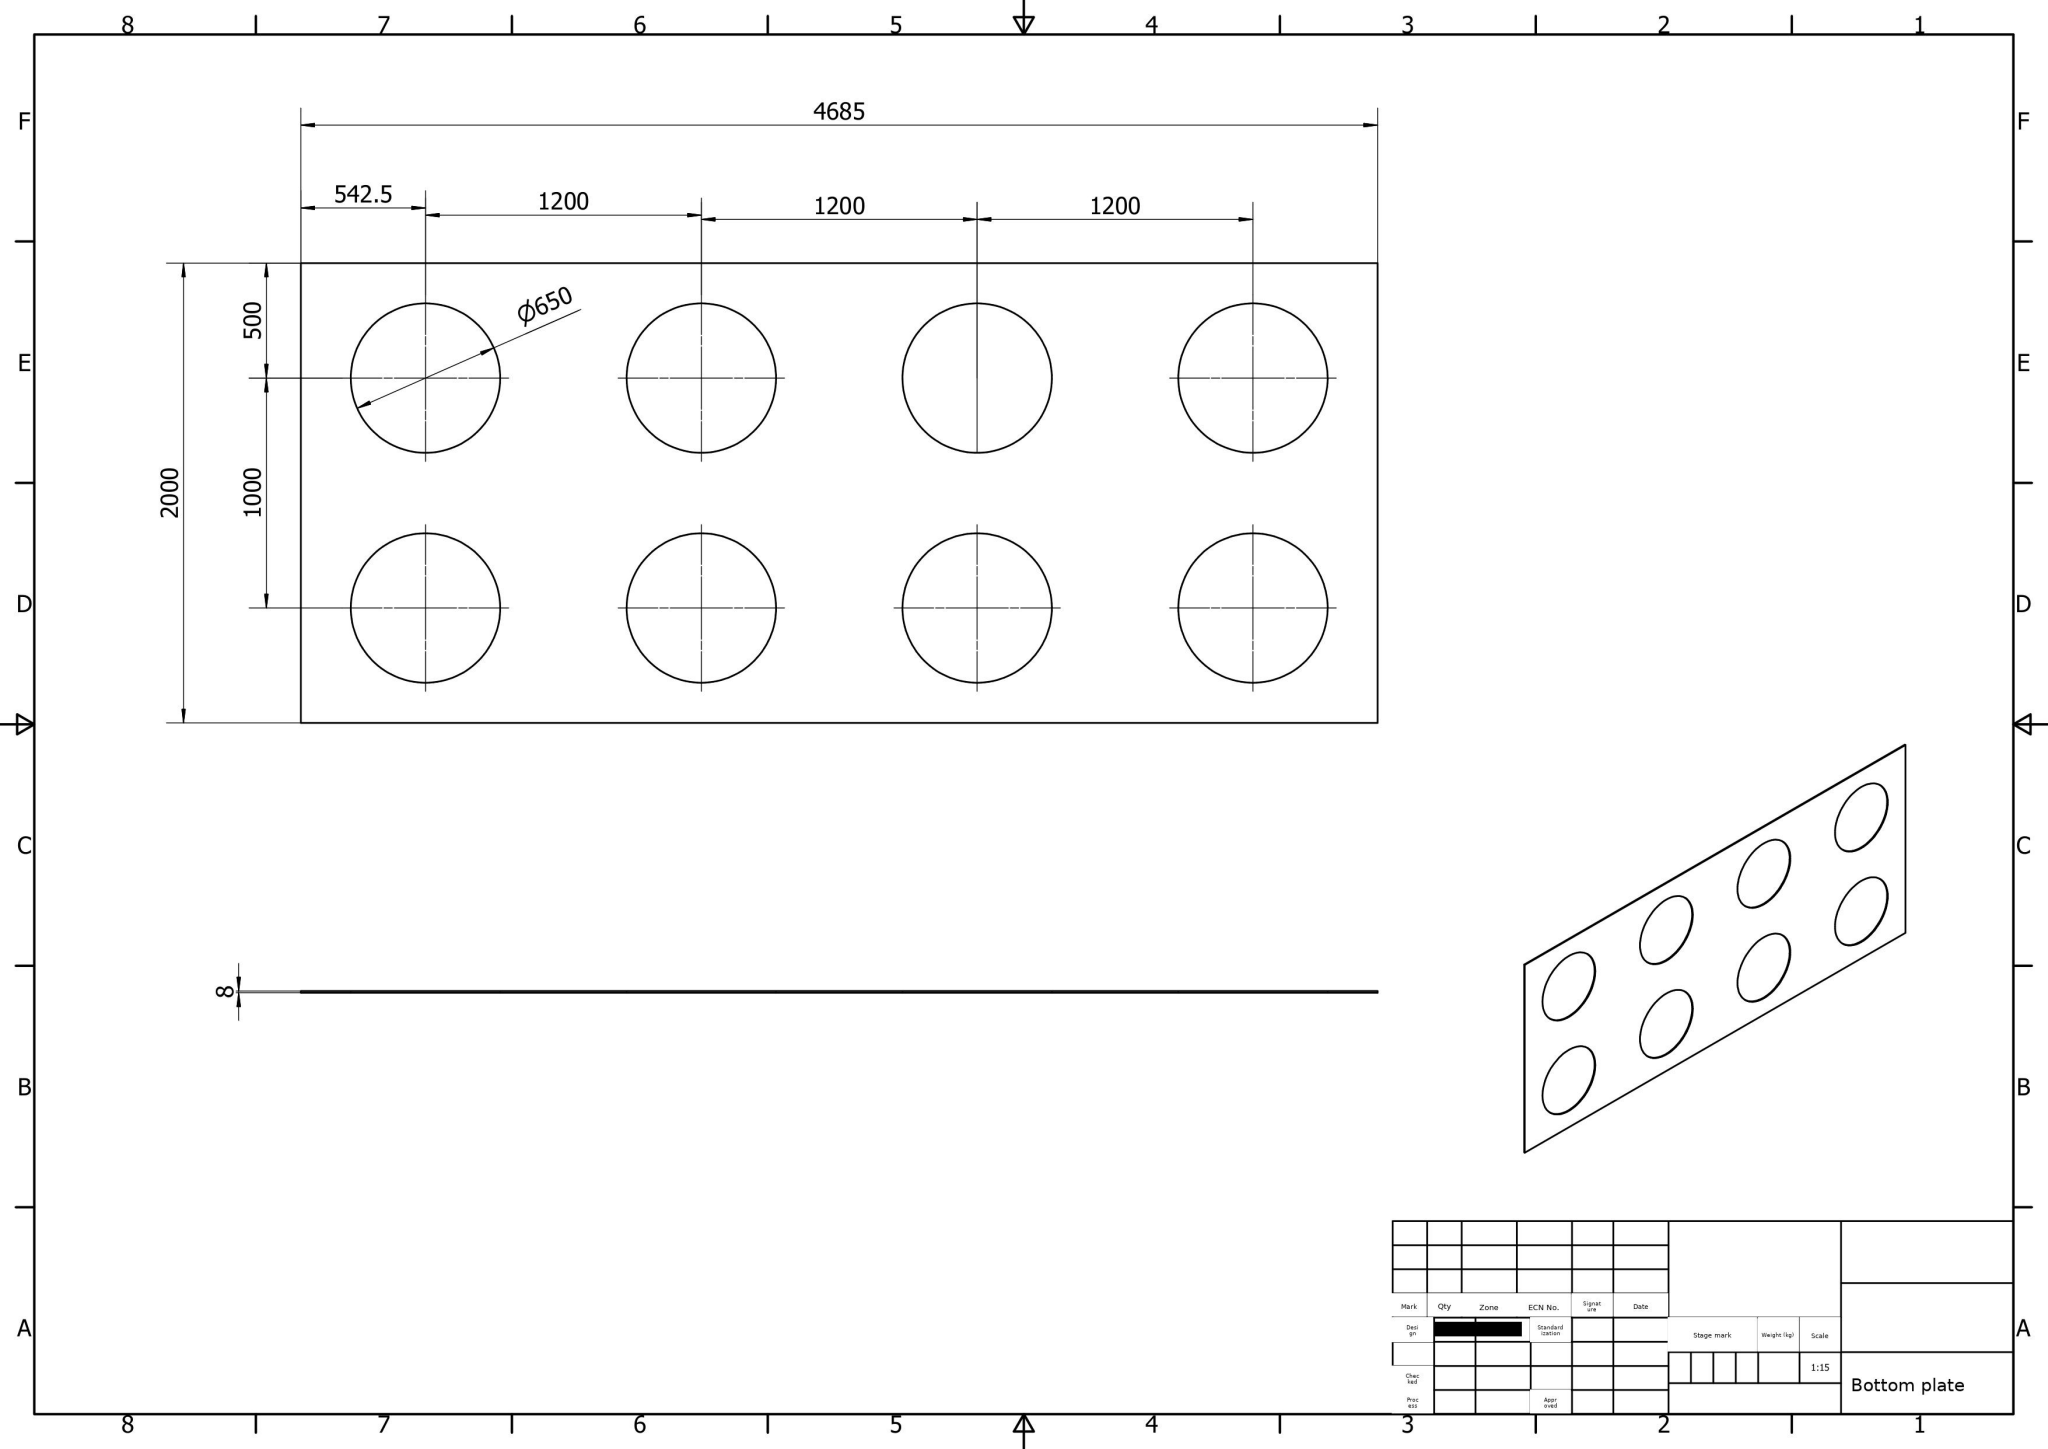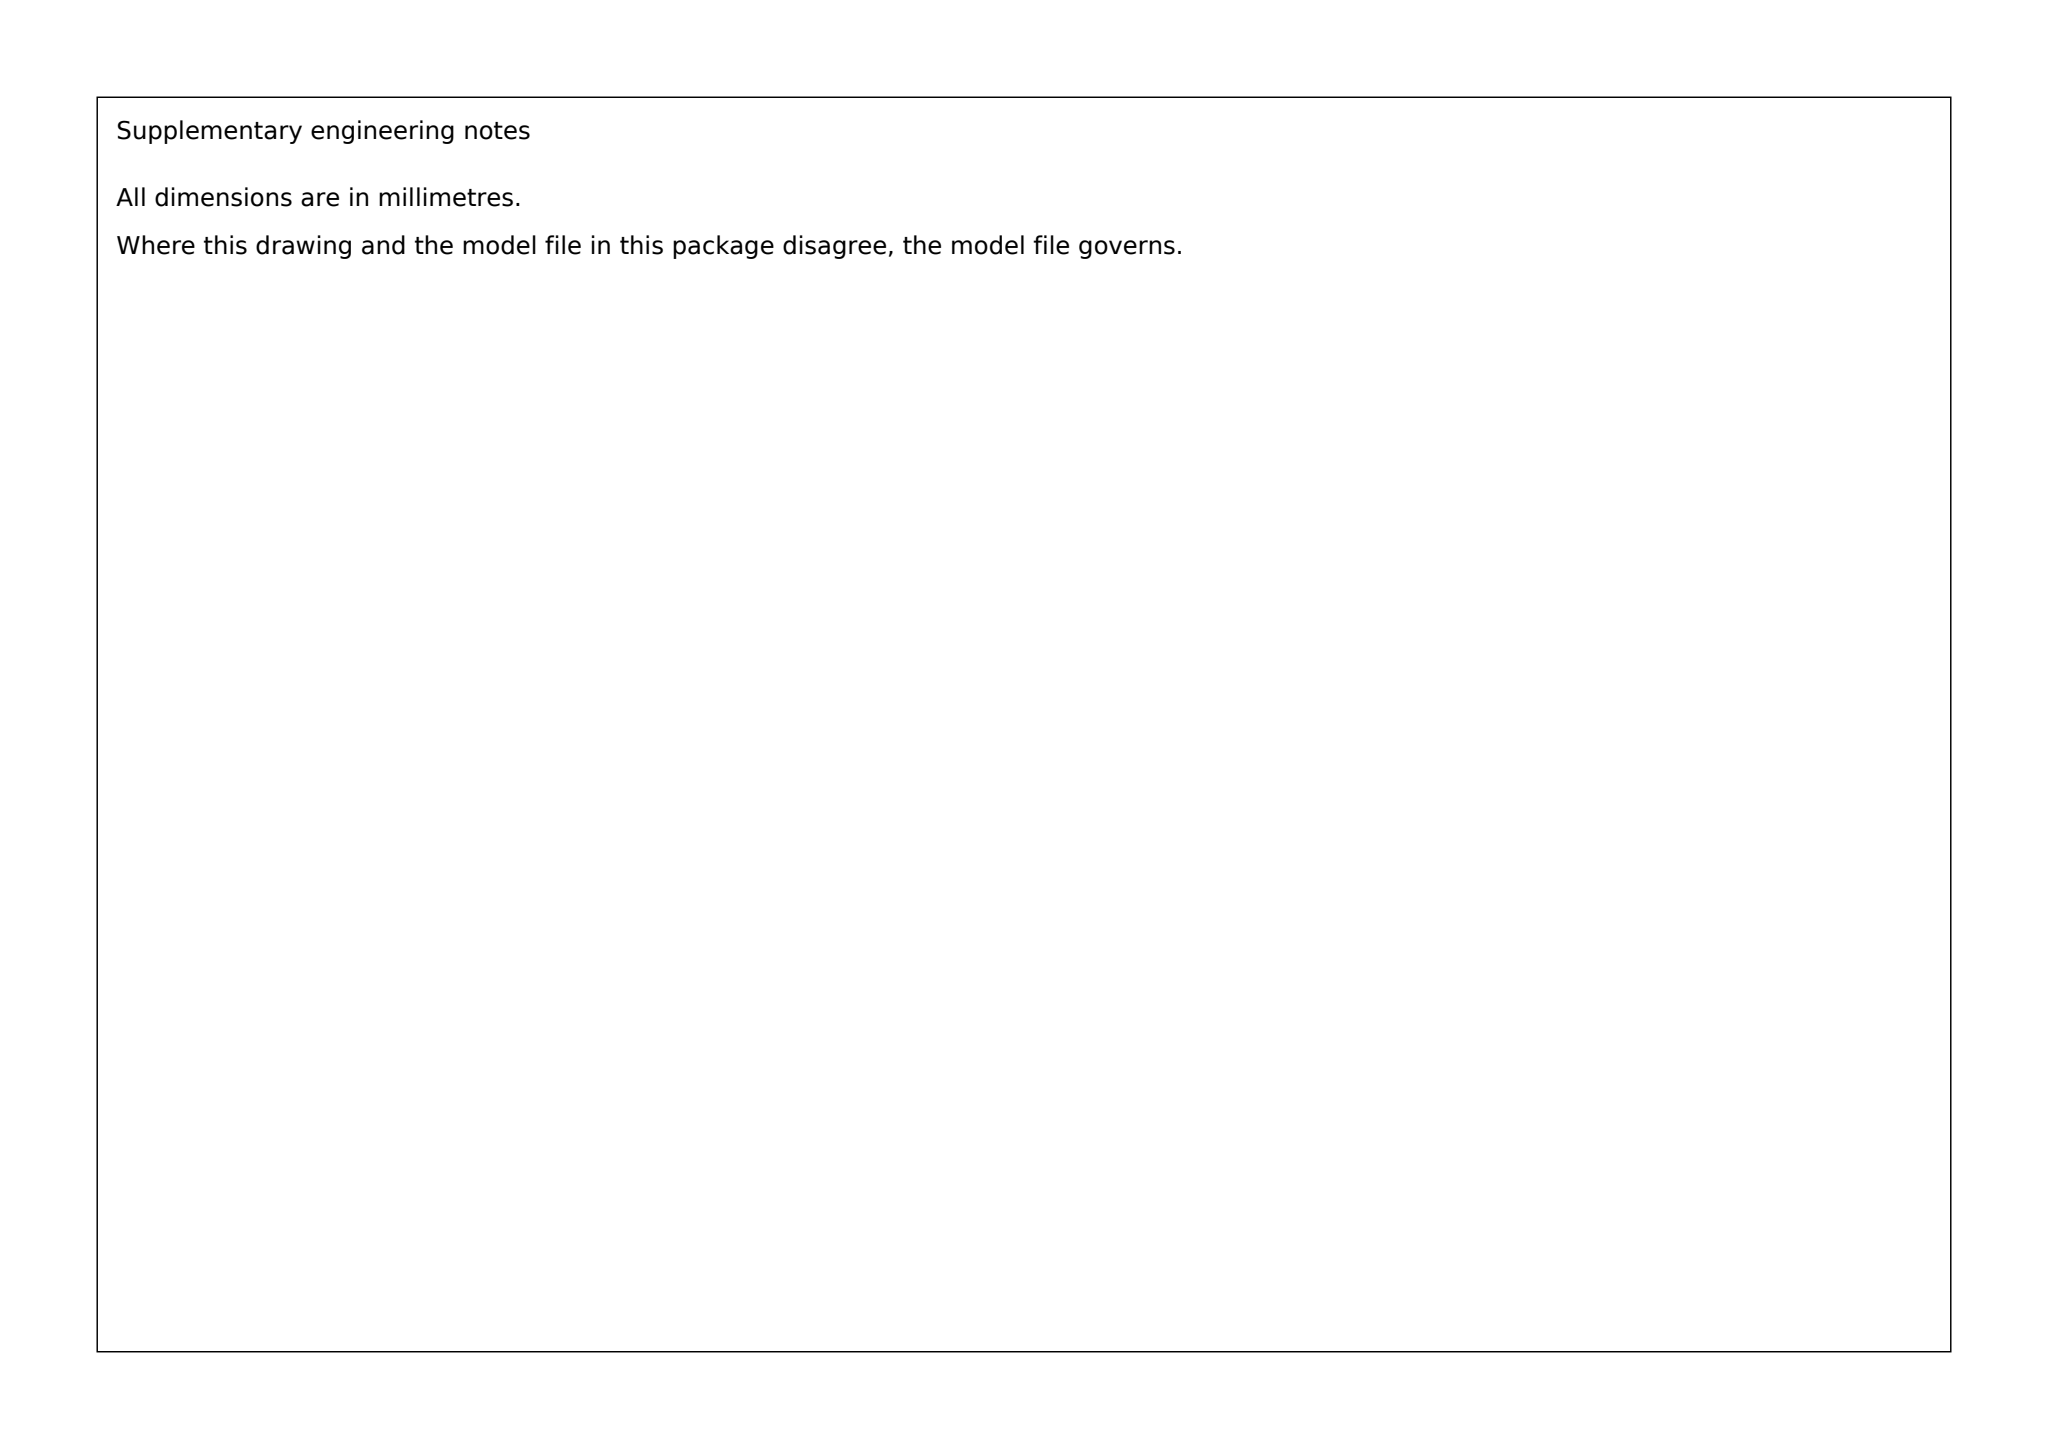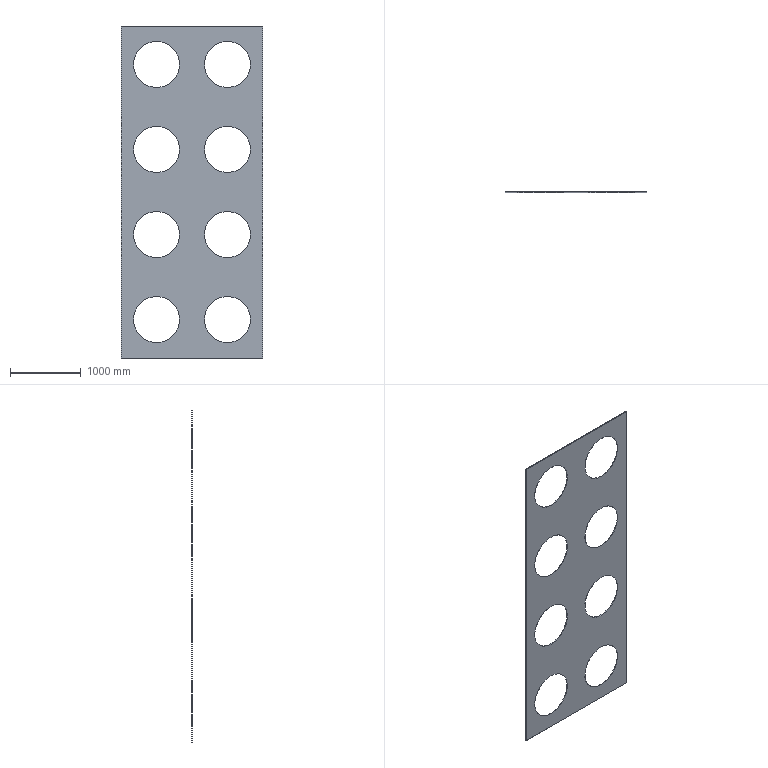Part | SolidWorks | mm | 1 solid | 22 faces | box 2000 x 8 x 4685 mm | volume 53722834 mm3 | cylinder 16 | plane 6 | commonest cylinder face diameters 650 x16
STEP:
#1=CARTESIAN_POINT('',(-500.,8.,2125.));
#2=VERTEX_POINT('',#1);
#3=CARTESIAN_POINT('',(-500.,8.,1475.));
#4=VERTEX_POINT('',#3);
#5=CARTESIAN_POINT('',(-500.,8.,1800.));
#6=DIRECTION('',(0.,-1.,0.));
#7=DIRECTION('',(0.,0.,-1.));
#8=AXIS2_PLACEMENT_3D('',#5,#6,#7);
#9=CIRCLE('',#8,325.);
#10=EDGE_CURVE('',#2,#4,#9,.T.);
#11=ORIENTED_EDGE('',*,*,#10,.F.);
#12=CARTESIAN_POINT('',(-500.,0.,2125.));
#13=VERTEX_POINT('',#12);
#14=CARTESIAN_POINT('',(-500.,8.,2125.));
#15=DIRECTION('',(0.,-1.,0.));
#16=VECTOR('',#15,1000.);
#17=LINE('',#14,#16);
#18=EDGE_CURVE('',#2,#13,#17,.T.);
#19=ORIENTED_EDGE('',*,*,#18,.T.);
#20=CARTESIAN_POINT('',(-500.,0.,1475.));
#21=VERTEX_POINT('',#20);
#22=CARTESIAN_POINT('',(-500.,0.,1800.));
#23=DIRECTION('',(0.,1.,0.));
#24=DIRECTION('',(0.,0.,-1.));
#25=AXIS2_PLACEMENT_3D('',#22,#23,#24);
#26=CIRCLE('',#25,325.);
#27=EDGE_CURVE('',#21,#13,#26,.T.);
#28=ORIENTED_EDGE('',*,*,#27,.F.);
#29=CARTESIAN_POINT('',(-500.,8.,1475.));
#30=DIRECTION('',(0.,-1.,0.));
#31=VECTOR('',#30,1000.);
#32=LINE('',#29,#31);
#33=EDGE_CURVE('',#4,#21,#32,.T.);
#34=ORIENTED_EDGE('',*,*,#33,.F.);
#35=EDGE_LOOP('',(#11,#19,#28,#34));
#36=FACE_OUTER_BOUND('',#35,.T.);
#37=CARTESIAN_POINT('',(-500.,8.,1800.));
#38=DIRECTION('',(0.,-1.,0.));
#39=DIRECTION('',(0.,0.,-1.));
#40=AXIS2_PLACEMENT_3D('',#37,#38,#39);
#41=CYLINDRICAL_SURFACE('',#40,325.);
#42=ADVANCED_FACE('',(#36),#41,.F.);
#43=CARTESIAN_POINT('',(-500.,8.,-1475.));
#44=VERTEX_POINT('',#43);
#45=CARTESIAN_POINT('',(-500.,8.,-2125.));
#46=VERTEX_POINT('',#45);
#47=CARTESIAN_POINT('',(-500.,8.,-1800.));
#48=DIRECTION('',(0.,-1.,0.));
#49=DIRECTION('',(0.,0.,-1.));
#50=AXIS2_PLACEMENT_3D('',#47,#48,#49);
#51=CIRCLE('',#50,325.);
#52=EDGE_CURVE('',#44,#46,#51,.T.);
#53=ORIENTED_EDGE('',*,*,#52,.F.);
#54=CARTESIAN_POINT('',(-500.,0.,-1475.));
#55=VERTEX_POINT('',#54);
#56=CARTESIAN_POINT('',(-500.,8.,-1475.));
#57=DIRECTION('',(0.,-1.,0.));
#58=VECTOR('',#57,1000.);
#59=LINE('',#56,#58);
#60=EDGE_CURVE('',#44,#55,#59,.T.);
#61=ORIENTED_EDGE('',*,*,#60,.T.);
#62=CARTESIAN_POINT('',(-500.,0.,-2125.));
#63=VERTEX_POINT('',#62);
#64=CARTESIAN_POINT('',(-500.,0.,-1800.));
#65=DIRECTION('',(0.,1.,0.));
#66=DIRECTION('',(0.,0.,-1.));
#67=AXIS2_PLACEMENT_3D('',#64,#65,#66);
#68=CIRCLE('',#67,325.);
#69=EDGE_CURVE('',#63,#55,#68,.T.);
#70=ORIENTED_EDGE('',*,*,#69,.F.);
#71=CARTESIAN_POINT('',(-500.,8.,-2125.));
#72=DIRECTION('',(0.,-1.,0.));
#73=VECTOR('',#72,1000.);
#74=LINE('',#71,#73);
#75=EDGE_CURVE('',#46,#63,#74,.T.);
#76=ORIENTED_EDGE('',*,*,#75,.F.);
#77=EDGE_LOOP('',(#53,#61,#70,#76));
#78=FACE_OUTER_BOUND('',#77,.T.);
#79=CARTESIAN_POINT('',(-500.,8.,-1800.));
#80=DIRECTION('',(0.,-1.,0.));
#81=DIRECTION('',(0.,0.,-1.));
#82=AXIS2_PLACEMENT_3D('',#79,#80,#81);
#83=CYLINDRICAL_SURFACE('',#82,325.);
#84=ADVANCED_FACE('',(#78),#83,.F.);
#85=CARTESIAN_POINT('',(-500.,8.,925.));
#86=VERTEX_POINT('',#85);
#87=CARTESIAN_POINT('',(-500.,8.,275.));
#88=VERTEX_POINT('',#87);
#89=CARTESIAN_POINT('',(-500.,8.,600.));
#90=DIRECTION('',(0.,-1.,0.));
#91=DIRECTION('',(0.,0.,-1.));
#92=AXIS2_PLACEMENT_3D('',#89,#90,#91);
#93=CIRCLE('',#92,325.);
#94=EDGE_CURVE('',#86,#88,#93,.T.);
#95=ORIENTED_EDGE('',*,*,#94,.F.);
#96=CARTESIAN_POINT('',(-500.,0.,925.));
#97=VERTEX_POINT('',#96);
#98=CARTESIAN_POINT('',(-500.,8.,925.));
#99=DIRECTION('',(0.,-1.,0.));
#100=VECTOR('',#99,1000.);
#101=LINE('',#98,#100);
#102=EDGE_CURVE('',#86,#97,#101,.T.);
#103=ORIENTED_EDGE('',*,*,#102,.T.);
#104=CARTESIAN_POINT('',(-500.,0.,275.));
#105=VERTEX_POINT('',#104);
#106=CARTESIAN_POINT('',(-500.,0.,600.));
#107=DIRECTION('',(0.,1.,0.));
#108=DIRECTION('',(0.,0.,-1.));
#109=AXIS2_PLACEMENT_3D('',#106,#107,#108);
#110=CIRCLE('',#109,325.);
#111=EDGE_CURVE('',#105,#97,#110,.T.);
#112=ORIENTED_EDGE('',*,*,#111,.F.);
#113=CARTESIAN_POINT('',(-500.,8.,275.));
#114=DIRECTION('',(0.,-1.,0.));
#115=VECTOR('',#114,1000.);
#116=LINE('',#113,#115);
#117=EDGE_CURVE('',#88,#105,#116,.T.);
#118=ORIENTED_EDGE('',*,*,#117,.F.);
#119=EDGE_LOOP('',(#95,#103,#112,#118));
#120=FACE_OUTER_BOUND('',#119,.T.);
#121=CARTESIAN_POINT('',(-500.,8.,600.));
#122=DIRECTION('',(0.,-1.,0.));
#123=DIRECTION('',(0.,0.,-1.));
#124=AXIS2_PLACEMENT_3D('',#121,#122,#123);
#125=CYLINDRICAL_SURFACE('',#124,325.);
#126=ADVANCED_FACE('',(#120),#125,.F.);
#127=CARTESIAN_POINT('',(-500.,8.,-275.));
#128=VERTEX_POINT('',#127);
#129=CARTESIAN_POINT('',(-500.,8.,-925.));
#130=VERTEX_POINT('',#129);
#131=CARTESIAN_POINT('',(-500.,8.,-600.));
#132=DIRECTION('',(0.,-1.,0.));
#133=DIRECTION('',(0.,0.,-1.));
#134=AXIS2_PLACEMENT_3D('',#131,#132,#133);
#135=CIRCLE('',#134,325.);
#136=EDGE_CURVE('',#128,#130,#135,.T.);
#137=ORIENTED_EDGE('',*,*,#136,.F.);
#138=CARTESIAN_POINT('',(-500.,0.,-275.));
#139=VERTEX_POINT('',#138);
#140=CARTESIAN_POINT('',(-500.,8.,-275.));
#141=DIRECTION('',(0.,-1.,0.));
#142=VECTOR('',#141,1000.);
#143=LINE('',#140,#142);
#144=EDGE_CURVE('',#128,#139,#143,.T.);
#145=ORIENTED_EDGE('',*,*,#144,.T.);
#146=CARTESIAN_POINT('',(-500.,0.,-925.));
#147=VERTEX_POINT('',#146);
#148=CARTESIAN_POINT('',(-500.,0.,-600.));
#149=DIRECTION('',(0.,1.,0.));
#150=DIRECTION('',(0.,0.,-1.));
#151=AXIS2_PLACEMENT_3D('',#148,#149,#150);
#152=CIRCLE('',#151,325.);
#153=EDGE_CURVE('',#147,#139,#152,.T.);
#154=ORIENTED_EDGE('',*,*,#153,.F.);
#155=CARTESIAN_POINT('',(-500.,8.,-925.));
#156=DIRECTION('',(0.,-1.,0.));
#157=VECTOR('',#156,1000.);
#158=LINE('',#155,#157);
#159=EDGE_CURVE('',#130,#147,#158,.T.);
#160=ORIENTED_EDGE('',*,*,#159,.F.);
#161=EDGE_LOOP('',(#137,#145,#154,#160));
#162=FACE_OUTER_BOUND('',#161,.T.);
#163=CARTESIAN_POINT('',(-500.,8.,-600.));
#164=DIRECTION('',(0.,-1.,0.));
#165=DIRECTION('',(0.,0.,-1.));
#166=AXIS2_PLACEMENT_3D('',#163,#164,#165);
#167=CYLINDRICAL_SURFACE('',#166,325.);
#168=ADVANCED_FACE('',(#162),#167,.F.);
#169=CARTESIAN_POINT('',(500.,0.,1475.));
#170=VERTEX_POINT('',#169);
#171=CARTESIAN_POINT('',(500.,0.,2125.));
#172=VERTEX_POINT('',#171);
#173=CARTESIAN_POINT('',(500.,0.,1800.));
#174=DIRECTION('',(0.,1.,0.));
#175=DIRECTION('',(0.,0.,1.));
#176=AXIS2_PLACEMENT_3D('',#173,#174,#175);
#177=CIRCLE('',#176,325.);
#178=EDGE_CURVE('',#170,#172,#177,.T.);
#179=ORIENTED_EDGE('',*,*,#178,.F.);
#180=CARTESIAN_POINT('',(500.,8.,1475.));
#181=VERTEX_POINT('',#180);
#182=CARTESIAN_POINT('',(500.,8.,1475.));
#183=DIRECTION('',(0.,1.,0.));
#184=VECTOR('',#183,1000.);
#185=LINE('',#182,#184);
#186=EDGE_CURVE('',#170,#181,#185,.T.);
#187=ORIENTED_EDGE('',*,*,#186,.T.);
#188=CARTESIAN_POINT('',(500.,8.,2125.));
#189=VERTEX_POINT('',#188);
#190=CARTESIAN_POINT('',(500.,8.,1800.));
#191=DIRECTION('',(0.,-1.,0.));
#192=DIRECTION('',(0.,0.,1.));
#193=AXIS2_PLACEMENT_3D('',#190,#191,#192);
#194=CIRCLE('',#193,325.);
#195=EDGE_CURVE('',#189,#181,#194,.T.);
#196=ORIENTED_EDGE('',*,*,#195,.F.);
#197=CARTESIAN_POINT('',(500.,8.,2125.));
#198=DIRECTION('',(0.,1.,0.));
#199=VECTOR('',#198,1000.);
#200=LINE('',#197,#199);
#201=EDGE_CURVE('',#172,#189,#200,.T.);
#202=ORIENTED_EDGE('',*,*,#201,.F.);
#203=EDGE_LOOP('',(#179,#187,#196,#202));
#204=FACE_OUTER_BOUND('',#203,.T.);
#205=CARTESIAN_POINT('',(500.,8.,1800.));
#206=DIRECTION('',(0.,1.,0.));
#207=DIRECTION('',(0.,0.,1.));
#208=AXIS2_PLACEMENT_3D('',#205,#206,#207);
#209=CYLINDRICAL_SURFACE('',#208,325.);
#210=ADVANCED_FACE('',(#204),#209,.F.);
#211=CARTESIAN_POINT('',(500.,0.,-2125.));
#212=VERTEX_POINT('',#211);
#213=CARTESIAN_POINT('',(500.,0.,-1475.));
#214=VERTEX_POINT('',#213);
#215=CARTESIAN_POINT('',(500.,0.,-1800.));
#216=DIRECTION('',(0.,1.,0.));
#217=DIRECTION('',(0.,0.,1.));
#218=AXIS2_PLACEMENT_3D('',#215,#216,#217);
#219=CIRCLE('',#218,325.);
#220=EDGE_CURVE('',#212,#214,#219,.T.);
#221=ORIENTED_EDGE('',*,*,#220,.F.);
#222=CARTESIAN_POINT('',(500.,8.,-2125.));
#223=VERTEX_POINT('',#222);
#224=CARTESIAN_POINT('',(500.,8.,-2125.));
#225=DIRECTION('',(0.,1.,0.));
#226=VECTOR('',#225,1000.);
#227=LINE('',#224,#226);
#228=EDGE_CURVE('',#212,#223,#227,.T.);
#229=ORIENTED_EDGE('',*,*,#228,.T.);
#230=CARTESIAN_POINT('',(500.,8.,-1475.));
#231=VERTEX_POINT('',#230);
#232=CARTESIAN_POINT('',(500.,8.,-1800.));
#233=DIRECTION('',(0.,-1.,0.));
#234=DIRECTION('',(0.,0.,1.));
#235=AXIS2_PLACEMENT_3D('',#232,#233,#234);
#236=CIRCLE('',#235,325.);
#237=EDGE_CURVE('',#231,#223,#236,.T.);
#238=ORIENTED_EDGE('',*,*,#237,.F.);
#239=CARTESIAN_POINT('',(500.,8.,-1475.));
#240=DIRECTION('',(0.,1.,0.));
#241=VECTOR('',#240,1000.);
#242=LINE('',#239,#241);
#243=EDGE_CURVE('',#214,#231,#242,.T.);
#244=ORIENTED_EDGE('',*,*,#243,.F.);
#245=EDGE_LOOP('',(#221,#229,#238,#244));
#246=FACE_OUTER_BOUND('',#245,.T.);
#247=CARTESIAN_POINT('',(500.,8.,-1800.));
#248=DIRECTION('',(0.,1.,0.));
#249=DIRECTION('',(0.,0.,1.));
#250=AXIS2_PLACEMENT_3D('',#247,#248,#249);
#251=CYLINDRICAL_SURFACE('',#250,325.);
#252=ADVANCED_FACE('',(#246),#251,.F.);
#253=CARTESIAN_POINT('',(500.,0.,275.));
#254=VERTEX_POINT('',#253);
#255=CARTESIAN_POINT('',(500.,0.,925.));
#256=VERTEX_POINT('',#255);
#257=CARTESIAN_POINT('',(500.,0.,600.));
#258=DIRECTION('',(0.,1.,0.));
#259=DIRECTION('',(0.,0.,1.));
#260=AXIS2_PLACEMENT_3D('',#257,#258,#259);
#261=CIRCLE('',#260,325.);
#262=EDGE_CURVE('',#254,#256,#261,.T.);
#263=ORIENTED_EDGE('',*,*,#262,.F.);
#264=CARTESIAN_POINT('',(500.,8.,275.));
#265=VERTEX_POINT('',#264);
#266=CARTESIAN_POINT('',(500.,8.,275.));
#267=DIRECTION('',(0.,1.,0.));
#268=VECTOR('',#267,1000.);
#269=LINE('',#266,#268);
#270=EDGE_CURVE('',#254,#265,#269,.T.);
#271=ORIENTED_EDGE('',*,*,#270,.T.);
#272=CARTESIAN_POINT('',(500.,8.,925.));
#273=VERTEX_POINT('',#272);
#274=CARTESIAN_POINT('',(500.,8.,600.));
#275=DIRECTION('',(0.,-1.,0.));
#276=DIRECTION('',(0.,0.,1.));
#277=AXIS2_PLACEMENT_3D('',#274,#275,#276);
#278=CIRCLE('',#277,325.);
#279=EDGE_CURVE('',#273,#265,#278,.T.);
#280=ORIENTED_EDGE('',*,*,#279,.F.);
#281=CARTESIAN_POINT('',(500.,8.,925.));
#282=DIRECTION('',(0.,1.,0.));
#283=VECTOR('',#282,1000.);
#284=LINE('',#281,#283);
#285=EDGE_CURVE('',#256,#273,#284,.T.);
#286=ORIENTED_EDGE('',*,*,#285,.F.);
#287=EDGE_LOOP('',(#263,#271,#280,#286));
#288=FACE_OUTER_BOUND('',#287,.T.);
#289=CARTESIAN_POINT('',(500.,8.,600.));
#290=DIRECTION('',(0.,1.,0.));
#291=DIRECTION('',(0.,0.,1.));
#292=AXIS2_PLACEMENT_3D('',#289,#290,#291);
#293=CYLINDRICAL_SURFACE('',#292,325.);
#294=ADVANCED_FACE('',(#288),#293,.F.);
#295=CARTESIAN_POINT('',(500.,0.,-925.));
#296=VERTEX_POINT('',#295);
#297=CARTESIAN_POINT('',(500.,0.,-275.));
#298=VERTEX_POINT('',#297);
#299=CARTESIAN_POINT('',(500.,0.,-600.));
#300=DIRECTION('',(0.,1.,0.));
#301=DIRECTION('',(0.,0.,1.));
#302=AXIS2_PLACEMENT_3D('',#299,#300,#301);
#303=CIRCLE('',#302,325.);
#304=EDGE_CURVE('',#296,#298,#303,.T.);
#305=ORIENTED_EDGE('',*,*,#304,.F.);
#306=CARTESIAN_POINT('',(500.,8.,-925.));
#307=VERTEX_POINT('',#306);
#308=CARTESIAN_POINT('',(500.,8.,-925.));
#309=DIRECTION('',(0.,1.,0.));
#310=VECTOR('',#309,1000.);
#311=LINE('',#308,#310);
#312=EDGE_CURVE('',#296,#307,#311,.T.);
#313=ORIENTED_EDGE('',*,*,#312,.T.);
#314=CARTESIAN_POINT('',(500.,8.,-275.));
#315=VERTEX_POINT('',#314);
#316=CARTESIAN_POINT('',(500.,8.,-600.));
#317=DIRECTION('',(0.,-1.,0.));
#318=DIRECTION('',(0.,0.,1.));
#319=AXIS2_PLACEMENT_3D('',#316,#317,#318);
#320=CIRCLE('',#319,325.);
#321=EDGE_CURVE('',#315,#307,#320,.T.);
#322=ORIENTED_EDGE('',*,*,#321,.F.);
#323=CARTESIAN_POINT('',(500.,8.,-275.));
#324=DIRECTION('',(0.,1.,0.));
#325=VECTOR('',#324,1000.);
#326=LINE('',#323,#325);
#327=EDGE_CURVE('',#298,#315,#326,.T.);
#328=ORIENTED_EDGE('',*,*,#327,.F.);
#329=EDGE_LOOP('',(#305,#313,#322,#328));
#330=FACE_OUTER_BOUND('',#329,.T.);
#331=CARTESIAN_POINT('',(500.,8.,-600.));
#332=DIRECTION('',(0.,1.,0.));
#333=DIRECTION('',(0.,0.,1.));
#334=AXIS2_PLACEMENT_3D('',#331,#332,#333);
#335=CYLINDRICAL_SURFACE('',#334,325.);
#336=ADVANCED_FACE('',(#330),#335,.F.);
#337=CARTESIAN_POINT('',(-500.,8.,1800.));
#338=DIRECTION('',(0.,-1.,0.));
#339=DIRECTION('',(0.,0.,-1.));
#340=AXIS2_PLACEMENT_3D('',#337,#338,#339);
#341=CIRCLE('',#340,325.);
#342=EDGE_CURVE('',#4,#2,#341,.T.);
#343=ORIENTED_EDGE('',*,*,#342,.T.);
#344=ORIENTED_EDGE('',*,*,#10,.T.);
#345=EDGE_LOOP('',(#343,#344));
#346=FACE_BOUND('',#345,.T.);
#347=CARTESIAN_POINT('',(-500.,8.,-1800.));
#348=DIRECTION('',(0.,-1.,0.));
#349=DIRECTION('',(0.,0.,-1.));
#350=AXIS2_PLACEMENT_3D('',#347,#348,#349);
#351=CIRCLE('',#350,325.);
#352=EDGE_CURVE('',#46,#44,#351,.T.);
#353=ORIENTED_EDGE('',*,*,#352,.T.);
#354=ORIENTED_EDGE('',*,*,#52,.T.);
#355=EDGE_LOOP('',(#353,#354));
#356=FACE_BOUND('',#355,.T.);
#357=CARTESIAN_POINT('',(-500.,8.,600.));
#358=DIRECTION('',(0.,-1.,0.));
#359=DIRECTION('',(0.,0.,-1.));
#360=AXIS2_PLACEMENT_3D('',#357,#358,#359);
#361=CIRCLE('',#360,325.);
#362=EDGE_CURVE('',#88,#86,#361,.T.);
#363=ORIENTED_EDGE('',*,*,#362,.T.);
#364=ORIENTED_EDGE('',*,*,#94,.T.);
#365=EDGE_LOOP('',(#363,#364));
#366=FACE_BOUND('',#365,.T.);
#367=CARTESIAN_POINT('',(-500.,8.,-600.));
#368=DIRECTION('',(0.,-1.,0.));
#369=DIRECTION('',(0.,0.,-1.));
#370=AXIS2_PLACEMENT_3D('',#367,#368,#369);
#371=CIRCLE('',#370,325.);
#372=EDGE_CURVE('',#130,#128,#371,.T.);
#373=ORIENTED_EDGE('',*,*,#372,.T.);
#374=ORIENTED_EDGE('',*,*,#136,.T.);
#375=EDGE_LOOP('',(#373,#374));
#376=FACE_BOUND('',#375,.T.);
#377=ORIENTED_EDGE('',*,*,#195,.T.);
#378=CARTESIAN_POINT('',(500.,8.,1800.));
#379=DIRECTION('',(0.,-1.,0.));
#380=DIRECTION('',(0.,0.,1.));
#381=AXIS2_PLACEMENT_3D('',#378,#379,#380);
#382=CIRCLE('',#381,325.);
#383=EDGE_CURVE('',#181,#189,#382,.T.);
#384=ORIENTED_EDGE('',*,*,#383,.T.);
#385=EDGE_LOOP('',(#377,#384));
#386=FACE_BOUND('',#385,.T.);
#387=ORIENTED_EDGE('',*,*,#237,.T.);
#388=CARTESIAN_POINT('',(500.,8.,-1800.));
#389=DIRECTION('',(0.,-1.,0.));
#390=DIRECTION('',(0.,0.,1.));
#391=AXIS2_PLACEMENT_3D('',#388,#389,#390);
#392=CIRCLE('',#391,325.);
#393=EDGE_CURVE('',#223,#231,#392,.T.);
#394=ORIENTED_EDGE('',*,*,#393,.T.);
#395=EDGE_LOOP('',(#387,#394));
#396=FACE_BOUND('',#395,.T.);
#397=ORIENTED_EDGE('',*,*,#279,.T.);
#398=CARTESIAN_POINT('',(500.,8.,600.));
#399=DIRECTION('',(0.,-1.,0.));
#400=DIRECTION('',(0.,0.,1.));
#401=AXIS2_PLACEMENT_3D('',#398,#399,#400);
#402=CIRCLE('',#401,325.);
#403=EDGE_CURVE('',#265,#273,#402,.T.);
#404=ORIENTED_EDGE('',*,*,#403,.T.);
#405=EDGE_LOOP('',(#397,#404));
#406=FACE_BOUND('',#405,.T.);
#407=ORIENTED_EDGE('',*,*,#321,.T.);
#408=CARTESIAN_POINT('',(500.,8.,-600.));
#409=DIRECTION('',(0.,-1.,0.));
#410=DIRECTION('',(0.,0.,1.));
#411=AXIS2_PLACEMENT_3D('',#408,#409,#410);
#412=CIRCLE('',#411,325.);
#413=EDGE_CURVE('',#307,#315,#412,.T.);
#414=ORIENTED_EDGE('',*,*,#413,.T.);
#415=EDGE_LOOP('',(#407,#414));
#416=FACE_BOUND('',#415,.T.);
#417=CARTESIAN_POINT('',(1000.,8.,-2342.5));
#418=VERTEX_POINT('',#417);
#419=CARTESIAN_POINT('',(-1000.,8.,-2342.5));
#420=VERTEX_POINT('',#419);
#421=CARTESIAN_POINT('',(0.,8.,-2342.5));
#422=DIRECTION('',(-1.,0.,0.));
#423=VECTOR('',#422,1000.);
#424=LINE('',#421,#423);
#425=EDGE_CURVE('',#418,#420,#424,.T.);
#426=ORIENTED_EDGE('',*,*,#425,.T.);
#427=CARTESIAN_POINT('',(-1000.,8.,2342.5));
#428=VERTEX_POINT('',#427);
#429=CARTESIAN_POINT('',(-1000.,8.,0.));
#430=DIRECTION('',(0.,0.,1.));
#431=VECTOR('',#430,1000.);
#432=LINE('',#429,#431);
#433=EDGE_CURVE('',#420,#428,#432,.T.);
#434=ORIENTED_EDGE('',*,*,#433,.T.);
#435=CARTESIAN_POINT('',(1000.,8.,2342.5));
#436=VERTEX_POINT('',#435);
#437=CARTESIAN_POINT('',(0.,8.,2342.5));
#438=DIRECTION('',(1.,0.,0.));
#439=VECTOR('',#438,1000.);
#440=LINE('',#437,#439);
#441=EDGE_CURVE('',#428,#436,#440,.T.);
#442=ORIENTED_EDGE('',*,*,#441,.T.);
#443=CARTESIAN_POINT('',(1000.,8.,0.));
#444=DIRECTION('',(0.,0.,-1.));
#445=VECTOR('',#444,1000.);
#446=LINE('',#443,#445);
#447=EDGE_CURVE('',#436,#418,#446,.T.);
#448=ORIENTED_EDGE('',*,*,#447,.T.);
#449=EDGE_LOOP('',(#426,#434,#442,#448));
#450=FACE_OUTER_BOUND('',#449,.T.);
#451=CARTESIAN_POINT('',(0.,8.,0.));
#452=DIRECTION('',(0.,1.,0.));
#453=DIRECTION('',(0.,0.,1.));
#454=AXIS2_PLACEMENT_3D('',#451,#452,#453);
#455=PLANE('',#454);
#456=ADVANCED_FACE('',(#346,#356,#366,#376,#386,#396,#406,#416,#450),#455,.T.);
#457=ORIENTED_EDGE('',*,*,#18,.F.);
#458=ORIENTED_EDGE('',*,*,#342,.F.);
#459=ORIENTED_EDGE('',*,*,#33,.T.);
#460=CARTESIAN_POINT('',(-500.,0.,1800.));
#461=DIRECTION('',(0.,1.,0.));
#462=DIRECTION('',(0.,0.,-1.));
#463=AXIS2_PLACEMENT_3D('',#460,#461,#462);
#464=CIRCLE('',#463,325.);
#465=EDGE_CURVE('',#13,#21,#464,.T.);
#466=ORIENTED_EDGE('',*,*,#465,.F.);
#467=EDGE_LOOP('',(#457,#458,#459,#466));
#468=FACE_OUTER_BOUND('',#467,.T.);
#469=CARTESIAN_POINT('',(-500.,8.,1800.));
#470=DIRECTION('',(0.,-1.,0.));
#471=DIRECTION('',(0.,0.,-1.));
#472=AXIS2_PLACEMENT_3D('',#469,#470,#471);
#473=CYLINDRICAL_SURFACE('',#472,325.);
#474=ADVANCED_FACE('',(#468),#473,.F.);
#475=ORIENTED_EDGE('',*,*,#60,.F.);
#476=ORIENTED_EDGE('',*,*,#352,.F.);
#477=ORIENTED_EDGE('',*,*,#75,.T.);
#478=CARTESIAN_POINT('',(-500.,0.,-1800.));
#479=DIRECTION('',(0.,1.,0.));
#480=DIRECTION('',(0.,0.,-1.));
#481=AXIS2_PLACEMENT_3D('',#478,#479,#480);
#482=CIRCLE('',#481,325.);
#483=EDGE_CURVE('',#55,#63,#482,.T.);
#484=ORIENTED_EDGE('',*,*,#483,.F.);
#485=EDGE_LOOP('',(#475,#476,#477,#484));
#486=FACE_OUTER_BOUND('',#485,.T.);
#487=CARTESIAN_POINT('',(-500.,8.,-1800.));
#488=DIRECTION('',(0.,-1.,0.));
#489=DIRECTION('',(0.,0.,-1.));
#490=AXIS2_PLACEMENT_3D('',#487,#488,#489);
#491=CYLINDRICAL_SURFACE('',#490,325.);
#492=ADVANCED_FACE('',(#486),#491,.F.);
#493=ORIENTED_EDGE('',*,*,#102,.F.);
#494=ORIENTED_EDGE('',*,*,#362,.F.);
#495=ORIENTED_EDGE('',*,*,#117,.T.);
#496=CARTESIAN_POINT('',(-500.,0.,600.));
#497=DIRECTION('',(0.,1.,0.));
#498=DIRECTION('',(0.,0.,-1.));
#499=AXIS2_PLACEMENT_3D('',#496,#497,#498);
#500=CIRCLE('',#499,325.);
#501=EDGE_CURVE('',#97,#105,#500,.T.);
#502=ORIENTED_EDGE('',*,*,#501,.F.);
#503=EDGE_LOOP('',(#493,#494,#495,#502));
#504=FACE_OUTER_BOUND('',#503,.T.);
#505=CARTESIAN_POINT('',(-500.,8.,600.));
#506=DIRECTION('',(0.,-1.,0.));
#507=DIRECTION('',(0.,0.,-1.));
#508=AXIS2_PLACEMENT_3D('',#505,#506,#507);
#509=CYLINDRICAL_SURFACE('',#508,325.);
#510=ADVANCED_FACE('',(#504),#509,.F.);
#511=ORIENTED_EDGE('',*,*,#144,.F.);
#512=ORIENTED_EDGE('',*,*,#372,.F.);
#513=ORIENTED_EDGE('',*,*,#159,.T.);
#514=CARTESIAN_POINT('',(-500.,0.,-600.));
#515=DIRECTION('',(0.,1.,0.));
#516=DIRECTION('',(0.,0.,-1.));
#517=AXIS2_PLACEMENT_3D('',#514,#515,#516);
#518=CIRCLE('',#517,325.);
#519=EDGE_CURVE('',#139,#147,#518,.T.);
#520=ORIENTED_EDGE('',*,*,#519,.F.);
#521=EDGE_LOOP('',(#511,#512,#513,#520));
#522=FACE_OUTER_BOUND('',#521,.T.);
#523=CARTESIAN_POINT('',(-500.,8.,-600.));
#524=DIRECTION('',(0.,-1.,0.));
#525=DIRECTION('',(0.,0.,-1.));
#526=AXIS2_PLACEMENT_3D('',#523,#524,#525);
#527=CYLINDRICAL_SURFACE('',#526,325.);
#528=ADVANCED_FACE('',(#522),#527,.F.);
#529=ORIENTED_EDGE('',*,*,#186,.F.);
#530=CARTESIAN_POINT('',(500.,0.,1800.));
#531=DIRECTION('',(0.,1.,0.));
#532=DIRECTION('',(0.,0.,1.));
#533=AXIS2_PLACEMENT_3D('',#530,#531,#532);
#534=CIRCLE('',#533,325.);
#535=EDGE_CURVE('',#172,#170,#534,.T.);
#536=ORIENTED_EDGE('',*,*,#535,.F.);
#537=ORIENTED_EDGE('',*,*,#201,.T.);
#538=ORIENTED_EDGE('',*,*,#383,.F.);
#539=EDGE_LOOP('',(#529,#536,#537,#538));
#540=FACE_OUTER_BOUND('',#539,.T.);
#541=CARTESIAN_POINT('',(500.,8.,1800.));
#542=DIRECTION('',(0.,1.,0.));
#543=DIRECTION('',(0.,0.,1.));
#544=AXIS2_PLACEMENT_3D('',#541,#542,#543);
#545=CYLINDRICAL_SURFACE('',#544,325.);
#546=ADVANCED_FACE('',(#540),#545,.F.);
#547=ORIENTED_EDGE('',*,*,#228,.F.);
#548=CARTESIAN_POINT('',(500.,0.,-1800.));
#549=DIRECTION('',(0.,1.,0.));
#550=DIRECTION('',(0.,0.,1.));
#551=AXIS2_PLACEMENT_3D('',#548,#549,#550);
#552=CIRCLE('',#551,325.);
#553=EDGE_CURVE('',#214,#212,#552,.T.);
#554=ORIENTED_EDGE('',*,*,#553,.F.);
#555=ORIENTED_EDGE('',*,*,#243,.T.);
#556=ORIENTED_EDGE('',*,*,#393,.F.);
#557=EDGE_LOOP('',(#547,#554,#555,#556));
#558=FACE_OUTER_BOUND('',#557,.T.);
#559=CARTESIAN_POINT('',(500.,8.,-1800.));
#560=DIRECTION('',(0.,1.,0.));
#561=DIRECTION('',(0.,0.,1.));
#562=AXIS2_PLACEMENT_3D('',#559,#560,#561);
#563=CYLINDRICAL_SURFACE('',#562,325.);
#564=ADVANCED_FACE('',(#558),#563,.F.);
#565=ORIENTED_EDGE('',*,*,#270,.F.);
#566=CARTESIAN_POINT('',(500.,0.,600.));
#567=DIRECTION('',(0.,1.,0.));
#568=DIRECTION('',(0.,0.,1.));
#569=AXIS2_PLACEMENT_3D('',#566,#567,#568);
#570=CIRCLE('',#569,325.);
#571=EDGE_CURVE('',#256,#254,#570,.T.);
#572=ORIENTED_EDGE('',*,*,#571,.F.);
#573=ORIENTED_EDGE('',*,*,#285,.T.);
#574=ORIENTED_EDGE('',*,*,#403,.F.);
#575=EDGE_LOOP('',(#565,#572,#573,#574));
#576=FACE_OUTER_BOUND('',#575,.T.);
#577=CARTESIAN_POINT('',(500.,8.,600.));
#578=DIRECTION('',(0.,1.,0.));
#579=DIRECTION('',(0.,0.,1.));
#580=AXIS2_PLACEMENT_3D('',#577,#578,#579);
#581=CYLINDRICAL_SURFACE('',#580,325.);
#582=ADVANCED_FACE('',(#576),#581,.F.);
#583=ORIENTED_EDGE('',*,*,#312,.F.);
#584=CARTESIAN_POINT('',(500.,0.,-600.));
#585=DIRECTION('',(0.,1.,0.));
#586=DIRECTION('',(0.,0.,1.));
#587=AXIS2_PLACEMENT_3D('',#584,#585,#586);
#588=CIRCLE('',#587,325.);
#589=EDGE_CURVE('',#298,#296,#588,.T.);
#590=ORIENTED_EDGE('',*,*,#589,.F.);
#591=ORIENTED_EDGE('',*,*,#327,.T.);
#592=ORIENTED_EDGE('',*,*,#413,.F.);
#593=EDGE_LOOP('',(#583,#590,#591,#592));
#594=FACE_OUTER_BOUND('',#593,.T.);
#595=CARTESIAN_POINT('',(500.,8.,-600.));
#596=DIRECTION('',(0.,1.,0.));
#597=DIRECTION('',(0.,0.,1.));
#598=AXIS2_PLACEMENT_3D('',#595,#596,#597);
#599=CYLINDRICAL_SURFACE('',#598,325.);
#600=ADVANCED_FACE('',(#594),#599,.F.);
#601=ORIENTED_EDGE('',*,*,#433,.F.);
#602=CARTESIAN_POINT('',(-1000.,0.,-2342.5));
#603=VERTEX_POINT('',#602);
#604=CARTESIAN_POINT('',(-1000.,0.,-2342.5));
#605=DIRECTION('',(0.,-1.,0.));
#606=VECTOR('',#605,1000.);
#607=LINE('',#604,#606);
#608=EDGE_CURVE('',#420,#603,#607,.T.);
#609=ORIENTED_EDGE('',*,*,#608,.T.);
#610=CARTESIAN_POINT('',(-1000.,0.,2342.5));
#611=VERTEX_POINT('',#610);
#612=CARTESIAN_POINT('',(-1000.,0.,-2342.5));
#613=DIRECTION('',(0.,0.,1.));
#614=VECTOR('',#613,1000.);
#615=LINE('',#612,#614);
#616=EDGE_CURVE('',#603,#611,#615,.T.);
#617=ORIENTED_EDGE('',*,*,#616,.T.);
#618=CARTESIAN_POINT('',(-1000.,0.,2342.5));
#619=DIRECTION('',(0.,1.,0.));
#620=VECTOR('',#619,1000.);
#621=LINE('',#618,#620);
#622=EDGE_CURVE('',#611,#428,#621,.T.);
#623=ORIENTED_EDGE('',*,*,#622,.T.);
#624=EDGE_LOOP('',(#601,#609,#617,#623));
#625=FACE_OUTER_BOUND('',#624,.T.);
#626=CARTESIAN_POINT('',(-1000.,0.,-2342.5));
#627=DIRECTION('',(-1.,0.,0.));
#628=DIRECTION('',(0.,0.,1.));
#629=AXIS2_PLACEMENT_3D('',#626,#627,#628);
#630=PLANE('',#629);
#631=ADVANCED_FACE('',(#625),#630,.T.);
#632=ORIENTED_EDGE('',*,*,#425,.F.);
#633=CARTESIAN_POINT('',(1000.,0.,-2342.5));
#634=VERTEX_POINT('',#633);
#635=CARTESIAN_POINT('',(1000.,0.,-2342.5));
#636=DIRECTION('',(0.,-1.,0.));
#637=VECTOR('',#636,1000.);
#638=LINE('',#635,#637);
#639=EDGE_CURVE('',#418,#634,#638,.T.);
#640=ORIENTED_EDGE('',*,*,#639,.T.);
#641=CARTESIAN_POINT('',(1000.,0.,-2342.5));
#642=DIRECTION('',(-1.,0.,0.));
#643=VECTOR('',#642,1000.);
#644=LINE('',#641,#643);
#645=EDGE_CURVE('',#634,#603,#644,.T.);
#646=ORIENTED_EDGE('',*,*,#645,.T.);
#647=ORIENTED_EDGE('',*,*,#608,.F.);
#648=EDGE_LOOP('',(#632,#640,#646,#647));
#649=FACE_OUTER_BOUND('',#648,.T.);
#650=CARTESIAN_POINT('',(1000.,0.,-2342.5));
#651=DIRECTION('',(0.,0.,-1.));
#652=DIRECTION('',(-1.,0.,0.));
#653=AXIS2_PLACEMENT_3D('',#650,#651,#652);
#654=PLANE('',#653);
#655=ADVANCED_FACE('',(#649),#654,.T.);
#656=ORIENTED_EDGE('',*,*,#447,.F.);
#657=CARTESIAN_POINT('',(1000.,0.,2342.5));
#658=VERTEX_POINT('',#657);
#659=CARTESIAN_POINT('',(1000.,0.,2342.5));
#660=DIRECTION('',(0.,-1.,0.));
#661=VECTOR('',#660,1000.);
#662=LINE('',#659,#661);
#663=EDGE_CURVE('',#436,#658,#662,.T.);
#664=ORIENTED_EDGE('',*,*,#663,.T.);
#665=CARTESIAN_POINT('',(1000.,0.,2342.5));
#666=DIRECTION('',(-0.,0.,-1.));
#667=VECTOR('',#666,1000.);
#668=LINE('',#665,#667);
#669=EDGE_CURVE('',#658,#634,#668,.T.);
#670=ORIENTED_EDGE('',*,*,#669,.T.);
#671=ORIENTED_EDGE('',*,*,#639,.F.);
#672=EDGE_LOOP('',(#656,#664,#670,#671));
#673=FACE_OUTER_BOUND('',#672,.T.);
#674=CARTESIAN_POINT('',(1000.,0.,2342.5));
#675=DIRECTION('',(1.,0.,-0.));
#676=DIRECTION('',(-0.,0.,-1.));
#677=AXIS2_PLACEMENT_3D('',#674,#675,#676);
#678=PLANE('',#677);
#679=ADVANCED_FACE('',(#673),#678,.T.);
#680=ORIENTED_EDGE('',*,*,#441,.F.);
#681=ORIENTED_EDGE('',*,*,#622,.F.);
#682=CARTESIAN_POINT('',(-1000.,0.,2342.5));
#683=DIRECTION('',(1.,0.,-0.));
#684=VECTOR('',#683,1000.);
#685=LINE('',#682,#684);
#686=EDGE_CURVE('',#611,#658,#685,.T.);
#687=ORIENTED_EDGE('',*,*,#686,.T.);
#688=ORIENTED_EDGE('',*,*,#663,.F.);
#689=EDGE_LOOP('',(#680,#681,#687,#688));
#690=FACE_OUTER_BOUND('',#689,.T.);
#691=CARTESIAN_POINT('',(-1000.,0.,2342.5));
#692=DIRECTION('',(0.,0.,1.));
#693=DIRECTION('',(1.,0.,-0.));
#694=AXIS2_PLACEMENT_3D('',#691,#692,#693);
#695=PLANE('',#694);
#696=ADVANCED_FACE('',(#690),#695,.T.);
#697=ORIENTED_EDGE('',*,*,#27,.T.);
#698=ORIENTED_EDGE('',*,*,#465,.T.);
#699=EDGE_LOOP('',(#697,#698));
#700=FACE_BOUND('',#699,.T.);
#701=ORIENTED_EDGE('',*,*,#69,.T.);
#702=ORIENTED_EDGE('',*,*,#483,.T.);
#703=EDGE_LOOP('',(#701,#702));
#704=FACE_BOUND('',#703,.T.);
#705=ORIENTED_EDGE('',*,*,#111,.T.);
#706=ORIENTED_EDGE('',*,*,#501,.T.);
#707=EDGE_LOOP('',(#705,#706));
#708=FACE_BOUND('',#707,.T.);
#709=ORIENTED_EDGE('',*,*,#153,.T.);
#710=ORIENTED_EDGE('',*,*,#519,.T.);
#711=EDGE_LOOP('',(#709,#710));
#712=FACE_BOUND('',#711,.T.);
#713=ORIENTED_EDGE('',*,*,#535,.T.);
#714=ORIENTED_EDGE('',*,*,#178,.T.);
#715=EDGE_LOOP('',(#713,#714));
#716=FACE_BOUND('',#715,.T.);
#717=ORIENTED_EDGE('',*,*,#553,.T.);
#718=ORIENTED_EDGE('',*,*,#220,.T.);
#719=EDGE_LOOP('',(#717,#718));
#720=FACE_BOUND('',#719,.T.);
#721=ORIENTED_EDGE('',*,*,#571,.T.);
#722=ORIENTED_EDGE('',*,*,#262,.T.);
#723=EDGE_LOOP('',(#721,#722));
#724=FACE_BOUND('',#723,.T.);
#725=ORIENTED_EDGE('',*,*,#589,.T.);
#726=ORIENTED_EDGE('',*,*,#304,.T.);
#727=EDGE_LOOP('',(#725,#726));
#728=FACE_BOUND('',#727,.T.);
#729=ORIENTED_EDGE('',*,*,#616,.F.);
#730=ORIENTED_EDGE('',*,*,#645,.F.);
#731=ORIENTED_EDGE('',*,*,#669,.F.);
#732=ORIENTED_EDGE('',*,*,#686,.F.);
#733=EDGE_LOOP('',(#729,#730,#731,#732));
#734=FACE_OUTER_BOUND('',#733,.T.);
#735=CARTESIAN_POINT('',(0.,0.,0.));
#736=DIRECTION('',(0.,1.,0.));
#737=DIRECTION('',(0.,0.,1.));
#738=AXIS2_PLACEMENT_3D('',#735,#736,#737);
#739=PLANE('',#738);
#740=ADVANCED_FACE('',(#700,#704,#708,#712,#716,#720,#724,#728,#734),#739,.F.);
#741=CLOSED_SHELL('',(#42,#84,#126,#168,#210,#252,#294,#336,#456,#474,#492,#510,#528,#546,#564,#582,#600,#631,#655,#679,#696,#740));
#742=MANIFOLD_SOLID_BREP('',#741);
#743=CARTESIAN_POINT('',(0.,0.,0.));
#744=DIRECTION('',(0.,0.,1.));
#745=DIRECTION('',(1.,0.,0.));
#746=AXIS2_PLACEMENT_3D('',#743,#744,#745);
#747=(LENGTH_UNIT()NAMED_UNIT(*)SI_UNIT(.MILLI.,.METRE.));
#748=UNCERTAINTY_MEASURE_WITH_UNIT(LENGTH_MEASURE(0.00001),#747,'','');
#749=(NAMED_UNIT(*)PLANE_ANGLE_UNIT()SI_UNIT($,.RADIAN.));
#750=(NAMED_UNIT(*)SI_UNIT($,.STERADIAN.)SOLID_ANGLE_UNIT());
#751=(GEOMETRIC_REPRESENTATION_CONTEXT(3)GLOBAL_UNCERTAINTY_ASSIGNED_CONTEXT((#748))GLOBAL_UNIT_ASSIGNED_CONTEXT((#747,#749,#750))REPRESENTATION_CONTEXT('',''));
#752=ADVANCED_BREP_SHAPE_REPRESENTATION('',(#742,#746),#751);